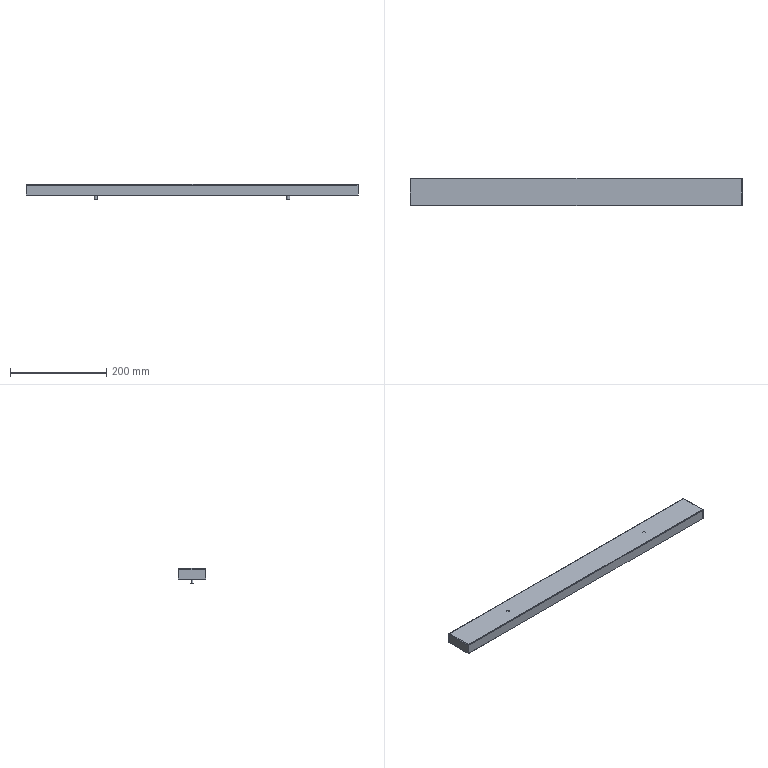Component | SolidWorks | KSHE-016.016-1 | 1 solid | 48 faces | volume 86393 mm3 | plane 36 | cylinder 12 | commonest cylinder face diameters 6 x4 2.6 x4 0.2 x4